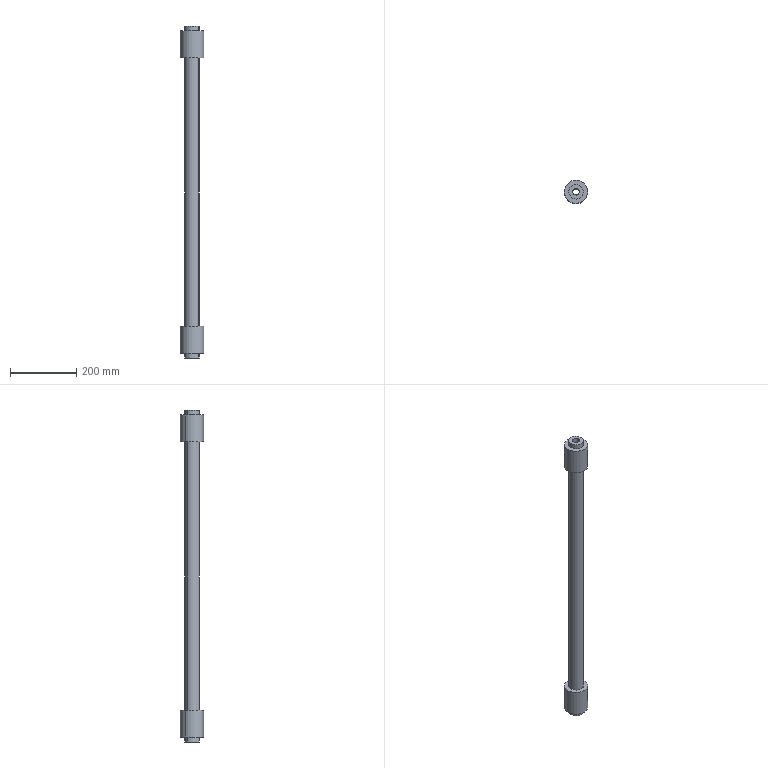Component | SolidWorks | Mandrel-1 | 1 solid | 18 faces | box 70 x 70 x 1000 mm | volume 1589826 mm3 | cylinder 12 | plane 6 | commonest cylinder face diameters 44.189 x6 70 x4 20 x2 | material 45
build123d program:
from build123d import *

# Parameters (mm, degrees)
SKETCH1_R           = 22.094
BOSS_EXTRUDE1_DEPTH = 1000
BOSS_EXTRUDE2_START = 15
SKETCH2_R           = 35
BOSS_EXTRUDE2_DEPTH = 80
SKETCH3_R           = 10
CUT_EXTRUDE1_DEPTH  = 1269.396


with BuildPart() as part:
    # Sketch1 → Boss-Extrude1 (new body)
    with BuildSketch(Plane.XY):
        with Locations((421.144, 598.058)):
            Circle(SKETCH1_R)
    extrude(amount=BOSS_EXTRUDE1_DEPTH)

    # Sketch2 → Boss-Extrude2 (add)
    with BuildSketch(Plane.XY.offset(BOSS_EXTRUDE2_START)):
        with Locations((421.144, 598.058)):
            Circle(SKETCH2_R)
    boss_extrude2 = extrude(amount=BOSS_EXTRUDE2_DEPTH)

    # Mirror1: Boss-Extrude2 across plane
    add(boss_extrude2.mirror(Plane.XY.offset(500)))

    # Sketch3 → Cut-Extrude1 (cut, through all)
    with BuildSketch(Plane(origin=(0, 0, 0), x_dir=(-1, 0, 0), z_dir=(0, 0, -1))):
        with Locations((-421.144, 598.058)):
            Circle(SKETCH3_R)
    extrude(amount=-CUT_EXTRUDE1_DEPTH, mode=Mode.SUBTRACT)


solid = part.part

# Placed as in the assembly
solid = solid.moved(Location((100, 0, -5), (0, 0, 0)))
STEP:
#1=COLOUR_RGB('',0.7922,0.8196,0.9333);
#2=FILL_AREA_STYLE_COLOUR('',#1);
#3=FILL_AREA_STYLE('',(#2));
#4=SURFACE_STYLE_FILL_AREA(#3);
#5=SURFACE_SIDE_STYLE('',(#4));
#6=SURFACE_STYLE_USAGE(.BOTH.,#5);
#7=PRESENTATION_STYLE_ASSIGNMENT((#6));
#8=CARTESIAN_POINT('',(20.191,23.766,39.173));
#9=VERTEX_POINT('',#8);
#10=CARTESIAN_POINT('',(20.844,23.325,39.173));
#11=VERTEX_POINT('',#10);
#12=CARTESIAN_POINT('',(20.517,23.546,39.173));
#13=DIRECTION('',(-0.,0.,-1.));
#14=DIRECTION('',(0.8284,-0.5601,0.));
#15=AXIS2_PLACEMENT_3D('',#12,#13,#14);
#16=CIRCLE('',#15,0.3937);
#17=EDGE_CURVE('',#9,#11,#16,.T.);
#18=ORIENTED_EDGE('',*,*,#17,.F.);
#19=CARTESIAN_POINT('',(20.191,23.766,-0.1969));
#20=VERTEX_POINT('',#19);
#21=CARTESIAN_POINT('',(20.191,23.766,39.173));
#22=DIRECTION('',(-0.,0.,-1.));
#23=VECTOR('',#22,39.37);
#24=LINE('',#21,#23);
#25=EDGE_CURVE('',#9,#20,#24,.T.);
#26=ORIENTED_EDGE('',*,*,#25,.T.);
#27=CARTESIAN_POINT('',(20.844,23.325,-0.1969));
#28=VERTEX_POINT('',#27);
#29=CARTESIAN_POINT('',(20.517,23.546,-0.1969));
#30=DIRECTION('',(-0.,0.,-1.));
#31=DIRECTION('',(0.8284,-0.5601,0.));
#32=AXIS2_PLACEMENT_3D('',#29,#30,#31);
#33=CIRCLE('',#32,0.3937);
#34=EDGE_CURVE('',#20,#28,#33,.T.);
#35=ORIENTED_EDGE('',*,*,#34,.T.);
#36=CARTESIAN_POINT('',(20.844,23.325,39.173));
#37=DIRECTION('',(-0.,0.,-1.));
#38=VECTOR('',#37,39.37);
#39=LINE('',#36,#38);
#40=EDGE_CURVE('',#11,#28,#39,.T.);
#41=ORIENTED_EDGE('',*,*,#40,.F.);
#42=EDGE_LOOP('',(#18,#26,#35,#41));
#43=FACE_OUTER_BOUND('',#42,.T.);
#44=CARTESIAN_POINT('',(20.517,23.546,39.173));
#45=DIRECTION('',(-0.,0.,-1.));
#46=DIRECTION('',(0.8284,-0.5601,0.));
#47=AXIS2_PLACEMENT_3D('',#44,#45,#46);
#48=CYLINDRICAL_SURFACE('',#47,0.3937);
#49=ADVANCED_FACE('',(#43),#48,.F.);
#50=CARTESIAN_POINT('',(19.797,24.033,39.173));
#51=VERTEX_POINT('',#50);
#52=CARTESIAN_POINT('',(21.238,23.058,39.173));
#53=VERTEX_POINT('',#52);
#54=CARTESIAN_POINT('',(20.517,23.546,39.173));
#55=DIRECTION('',(0.,-0.,1.));
#56=DIRECTION('',(-0.8284,0.5601,0.));
#57=AXIS2_PLACEMENT_3D('',#54,#55,#56);
#58=CIRCLE('',#57,0.8699);
#59=EDGE_CURVE('',#51,#53,#58,.T.);
#60=ORIENTED_EDGE('',*,*,#59,.F.);
#61=CARTESIAN_POINT('',(19.797,24.033,38.583));
#62=VERTEX_POINT('',#61);
#63=CARTESIAN_POINT('',(19.797,24.033,39.173));
#64=DIRECTION('',(-0.,0.,-1.));
#65=VECTOR('',#64,39.37);
#66=LINE('',#63,#65);
#67=EDGE_CURVE('',#51,#62,#66,.T.);
#68=ORIENTED_EDGE('',*,*,#67,.T.);
#69=CARTESIAN_POINT('',(21.238,23.058,38.583));
#70=VERTEX_POINT('',#69);
#71=CARTESIAN_POINT('',(20.517,23.546,38.583));
#72=DIRECTION('',(-0.,0.,-1.));
#73=DIRECTION('',(0.8284,-0.5601,0.));
#74=AXIS2_PLACEMENT_3D('',#71,#72,#73);
#75=CIRCLE('',#74,0.8699);
#76=EDGE_CURVE('',#70,#62,#75,.T.);
#77=ORIENTED_EDGE('',*,*,#76,.F.);
#78=CARTESIAN_POINT('',(21.238,23.058,39.173));
#79=DIRECTION('',(-0.,0.,-1.));
#80=VECTOR('',#79,39.37);
#81=LINE('',#78,#80);
#82=EDGE_CURVE('',#53,#70,#81,.T.);
#83=ORIENTED_EDGE('',*,*,#82,.F.);
#84=EDGE_LOOP('',(#60,#68,#77,#83));
#85=FACE_OUTER_BOUND('',#84,.T.);
#86=CARTESIAN_POINT('',(20.517,23.546,39.173));
#87=DIRECTION('',(-0.,0.,-1.));
#88=DIRECTION('',(0.8284,-0.5601,0.));
#89=AXIS2_PLACEMENT_3D('',#86,#87,#88);
#90=CYLINDRICAL_SURFACE('',#89,0.8699);
#91=ADVANCED_FACE('',(#85),#90,.T.);
#92=CARTESIAN_POINT('',(19.376,24.317,35.433));
#93=VERTEX_POINT('',#92);
#94=CARTESIAN_POINT('',(21.659,22.774,35.433));
#95=VERTEX_POINT('',#94);
#96=CARTESIAN_POINT('',(20.517,23.546,35.433));
#97=DIRECTION('',(0.,-0.,1.));
#98=DIRECTION('',(-0.8284,0.5601,0.));
#99=AXIS2_PLACEMENT_3D('',#96,#97,#98);
#100=CIRCLE('',#99,1.378);
#101=EDGE_CURVE('',#93,#95,#100,.T.);
#102=ORIENTED_EDGE('',*,*,#101,.T.);
#103=CARTESIAN_POINT('',(21.659,22.774,38.583));
#104=VERTEX_POINT('',#103);
#105=CARTESIAN_POINT('',(21.659,22.774,35.433));
#106=DIRECTION('',(0.,-0.,1.));
#107=VECTOR('',#106,39.37);
#108=LINE('',#105,#107);
#109=EDGE_CURVE('',#95,#104,#108,.T.);
#110=ORIENTED_EDGE('',*,*,#109,.T.);
#111=CARTESIAN_POINT('',(19.376,24.317,38.583));
#112=VERTEX_POINT('',#111);
#113=CARTESIAN_POINT('',(20.517,23.546,38.583));
#114=DIRECTION('',(0.,-0.,1.));
#115=DIRECTION('',(-0.8284,0.5601,0.));
#116=AXIS2_PLACEMENT_3D('',#113,#114,#115);
#117=CIRCLE('',#116,1.378);
#118=EDGE_CURVE('',#112,#104,#117,.T.);
#119=ORIENTED_EDGE('',*,*,#118,.F.);
#120=CARTESIAN_POINT('',(19.376,24.317,35.433));
#121=DIRECTION('',(0.,-0.,1.));
#122=VECTOR('',#121,39.37);
#123=LINE('',#120,#122);
#124=EDGE_CURVE('',#93,#112,#123,.T.);
#125=ORIENTED_EDGE('',*,*,#124,.F.);
#126=EDGE_LOOP('',(#102,#110,#119,#125));
#127=FACE_OUTER_BOUND('',#126,.T.);
#128=CARTESIAN_POINT('',(20.517,23.546,35.433));
#129=DIRECTION('',(0.,-0.,1.));
#130=DIRECTION('',(-0.8284,0.5601,0.));
#131=AXIS2_PLACEMENT_3D('',#128,#129,#130);
#132=CYLINDRICAL_SURFACE('',#131,1.378);
#133=ADVANCED_FACE('',(#127),#132,.T.);
#134=CARTESIAN_POINT('',(19.797,24.033,0.3937));
#135=VERTEX_POINT('',#134);
#136=CARTESIAN_POINT('',(21.238,23.058,0.3937));
#137=VERTEX_POINT('',#136);
#138=CARTESIAN_POINT('',(20.517,23.546,0.3937));
#139=DIRECTION('',(0.,-0.,1.));
#140=DIRECTION('',(-0.8284,0.5601,0.));
#141=AXIS2_PLACEMENT_3D('',#138,#139,#140);
#142=CIRCLE('',#141,0.8699);
#143=EDGE_CURVE('',#135,#137,#142,.T.);
#144=ORIENTED_EDGE('',*,*,#143,.F.);
#145=CARTESIAN_POINT('',(19.797,24.033,-0.1969));
#146=VERTEX_POINT('',#145);
#147=CARTESIAN_POINT('',(19.797,24.033,39.173));
#148=DIRECTION('',(-0.,0.,-1.));
#149=VECTOR('',#148,39.37);
#150=LINE('',#147,#149);
#151=EDGE_CURVE('',#135,#146,#150,.T.);
#152=ORIENTED_EDGE('',*,*,#151,.T.);
#153=CARTESIAN_POINT('',(21.238,23.058,-0.1969));
#154=VERTEX_POINT('',#153);
#155=CARTESIAN_POINT('',(20.517,23.546,-0.1969));
#156=DIRECTION('',(0.,-0.,1.));
#157=DIRECTION('',(-0.8284,0.5601,0.));
#158=AXIS2_PLACEMENT_3D('',#155,#156,#157);
#159=CIRCLE('',#158,0.8699);
#160=EDGE_CURVE('',#146,#154,#159,.T.);
#161=ORIENTED_EDGE('',*,*,#160,.T.);
#162=CARTESIAN_POINT('',(21.238,23.058,39.173));
#163=DIRECTION('',(-0.,0.,-1.));
#164=VECTOR('',#163,39.37);
#165=LINE('',#162,#164);
#166=EDGE_CURVE('',#137,#154,#165,.T.);
#167=ORIENTED_EDGE('',*,*,#166,.F.);
#168=EDGE_LOOP('',(#144,#152,#161,#167));
#169=FACE_OUTER_BOUND('',#168,.T.);
#170=CARTESIAN_POINT('',(20.517,23.546,39.173));
#171=DIRECTION('',(-0.,0.,-1.));
#172=DIRECTION('',(0.8284,-0.5601,0.));
#173=AXIS2_PLACEMENT_3D('',#170,#171,#172);
#174=CYLINDRICAL_SURFACE('',#173,0.8699);
#175=ADVANCED_FACE('',(#169),#174,.T.);
#176=CARTESIAN_POINT('',(19.376,24.317,3.543));
#177=VERTEX_POINT('',#176);
#178=CARTESIAN_POINT('',(21.659,22.774,3.543));
#179=VERTEX_POINT('',#178);
#180=CARTESIAN_POINT('',(20.517,23.546,3.543));
#181=DIRECTION('',(0.,-0.,1.));
#182=DIRECTION('',(-0.8284,0.5601,0.));
#183=AXIS2_PLACEMENT_3D('',#180,#181,#182);
#184=CIRCLE('',#183,1.378);
#185=EDGE_CURVE('',#177,#179,#184,.T.);
#186=ORIENTED_EDGE('',*,*,#185,.F.);
#187=CARTESIAN_POINT('',(19.376,24.317,0.3937));
#188=VERTEX_POINT('',#187);
#189=CARTESIAN_POINT('',(19.376,24.317,3.543));
#190=DIRECTION('',(-0.,0.,-1.));
#191=VECTOR('',#190,39.37);
#192=LINE('',#189,#191);
#193=EDGE_CURVE('',#177,#188,#192,.T.);
#194=ORIENTED_EDGE('',*,*,#193,.T.);
#195=CARTESIAN_POINT('',(21.659,22.774,0.3937));
#196=VERTEX_POINT('',#195);
#197=CARTESIAN_POINT('',(20.517,23.546,0.3937));
#198=DIRECTION('',(0.,-0.,1.));
#199=DIRECTION('',(-0.8284,0.5601,0.));
#200=AXIS2_PLACEMENT_3D('',#197,#198,#199);
#201=CIRCLE('',#200,1.378);
#202=EDGE_CURVE('',#188,#196,#201,.T.);
#203=ORIENTED_EDGE('',*,*,#202,.T.);
#204=CARTESIAN_POINT('',(21.659,22.774,3.543));
#205=DIRECTION('',(-0.,0.,-1.));
#206=VECTOR('',#205,39.37);
#207=LINE('',#204,#206);
#208=EDGE_CURVE('',#179,#196,#207,.T.);
#209=ORIENTED_EDGE('',*,*,#208,.F.);
#210=EDGE_LOOP('',(#186,#194,#203,#209));
#211=FACE_OUTER_BOUND('',#210,.T.);
#212=CARTESIAN_POINT('',(20.517,23.546,3.543));
#213=DIRECTION('',(-0.,0.,-1.));
#214=DIRECTION('',(0.8284,-0.5601,0.));
#215=AXIS2_PLACEMENT_3D('',#212,#213,#214);
#216=CYLINDRICAL_SURFACE('',#215,1.378);
#217=ADVANCED_FACE('',(#211),#216,.T.);
#218=CARTESIAN_POINT('',(21.238,23.058,35.433));
#219=VERTEX_POINT('',#218);
#220=CARTESIAN_POINT('',(19.797,24.033,35.433));
#221=VERTEX_POINT('',#220);
#222=CARTESIAN_POINT('',(20.517,23.546,35.433));
#223=DIRECTION('',(-0.,0.,-1.));
#224=DIRECTION('',(0.8284,-0.5601,0.));
#225=AXIS2_PLACEMENT_3D('',#222,#223,#224);
#226=CIRCLE('',#225,0.8699);
#227=EDGE_CURVE('',#219,#221,#226,.T.);
#228=ORIENTED_EDGE('',*,*,#227,.T.);
#229=CARTESIAN_POINT('',(19.797,24.033,3.543));
#230=VERTEX_POINT('',#229);
#231=CARTESIAN_POINT('',(19.797,24.033,39.173));
#232=DIRECTION('',(-0.,0.,-1.));
#233=VECTOR('',#232,39.37);
#234=LINE('',#231,#233);
#235=EDGE_CURVE('',#221,#230,#234,.T.);
#236=ORIENTED_EDGE('',*,*,#235,.T.);
#237=CARTESIAN_POINT('',(21.238,23.058,3.543));
#238=VERTEX_POINT('',#237);
#239=CARTESIAN_POINT('',(20.517,23.546,3.543));
#240=DIRECTION('',(0.,-0.,1.));
#241=DIRECTION('',(-0.8284,0.5601,0.));
#242=AXIS2_PLACEMENT_3D('',#239,#240,#241);
#243=CIRCLE('',#242,0.8699);
#244=EDGE_CURVE('',#230,#238,#243,.T.);
#245=ORIENTED_EDGE('',*,*,#244,.T.);
#246=CARTESIAN_POINT('',(21.238,23.058,39.173));
#247=DIRECTION('',(-0.,0.,-1.));
#248=VECTOR('',#247,39.37);
#249=LINE('',#246,#248);
#250=EDGE_CURVE('',#219,#238,#249,.T.);
#251=ORIENTED_EDGE('',*,*,#250,.F.);
#252=EDGE_LOOP('',(#228,#236,#245,#251));
#253=FACE_OUTER_BOUND('',#252,.T.);
#254=CARTESIAN_POINT('',(20.517,23.546,39.173));
#255=DIRECTION('',(-0.,0.,-1.));
#256=DIRECTION('',(0.8284,-0.5601,0.));
#257=AXIS2_PLACEMENT_3D('',#254,#255,#256);
#258=CYLINDRICAL_SURFACE('',#257,0.8699);
#259=ADVANCED_FACE('',(#253),#258,.T.);
#260=ORIENTED_EDGE('',*,*,#235,.F.);
#261=CARTESIAN_POINT('',(20.517,23.546,35.433));
#262=DIRECTION('',(-0.,0.,-1.));
#263=DIRECTION('',(0.8284,-0.5601,0.));
#264=AXIS2_PLACEMENT_3D('',#261,#262,#263);
#265=CIRCLE('',#264,0.8699);
#266=EDGE_CURVE('',#221,#219,#265,.T.);
#267=ORIENTED_EDGE('',*,*,#266,.T.);
#268=ORIENTED_EDGE('',*,*,#250,.T.);
#269=CARTESIAN_POINT('',(20.517,23.546,3.543));
#270=DIRECTION('',(0.,-0.,1.));
#271=DIRECTION('',(-0.8284,0.5601,0.));
#272=AXIS2_PLACEMENT_3D('',#269,#270,#271);
#273=CIRCLE('',#272,0.8699);
#274=EDGE_CURVE('',#238,#230,#273,.T.);
#275=ORIENTED_EDGE('',*,*,#274,.T.);
#276=EDGE_LOOP('',(#260,#267,#268,#275));
#277=FACE_OUTER_BOUND('',#276,.T.);
#278=CARTESIAN_POINT('',(20.517,23.546,39.173));
#279=DIRECTION('',(-0.,0.,-1.));
#280=DIRECTION('',(0.8284,-0.5601,0.));
#281=AXIS2_PLACEMENT_3D('',#278,#279,#280);
#282=CYLINDRICAL_SURFACE('',#281,0.8699);
#283=ADVANCED_FACE('',(#277),#282,.T.);
#284=CARTESIAN_POINT('',(20.517,23.546,3.543));
#285=DIRECTION('',(0.,-0.,1.));
#286=DIRECTION('',(-0.8284,0.5601,0.));
#287=AXIS2_PLACEMENT_3D('',#284,#285,#286);
#288=CIRCLE('',#287,1.378);
#289=EDGE_CURVE('',#179,#177,#288,.T.);
#290=ORIENTED_EDGE('',*,*,#289,.T.);
#291=ORIENTED_EDGE('',*,*,#185,.T.);
#292=EDGE_LOOP('',(#290,#291));
#293=FACE_OUTER_BOUND('',#292,.T.);
#294=ORIENTED_EDGE('',*,*,#274,.F.);
#295=ORIENTED_EDGE('',*,*,#244,.F.);
#296=EDGE_LOOP('',(#294,#295));
#297=FACE_BOUND('',#296,.T.);
#298=CARTESIAN_POINT('',(20.517,23.546,3.543));
#299=DIRECTION('',(0.,-0.,1.));
#300=DIRECTION('',(-0.8284,0.5601,0.));
#301=AXIS2_PLACEMENT_3D('',#298,#299,#300);
#302=PLANE('',#301);
#303=ADVANCED_FACE('',(#293,#297),#302,.T.);
#304=CARTESIAN_POINT('',(20.517,23.546,0.3937));
#305=DIRECTION('',(0.,-0.,1.));
#306=DIRECTION('',(-0.8284,0.5601,0.));
#307=AXIS2_PLACEMENT_3D('',#304,#305,#306);
#308=CIRCLE('',#307,1.378);
#309=EDGE_CURVE('',#196,#188,#308,.T.);
#310=ORIENTED_EDGE('',*,*,#309,.F.);
#311=ORIENTED_EDGE('',*,*,#202,.F.);
#312=EDGE_LOOP('',(#310,#311));
#313=FACE_OUTER_BOUND('',#312,.T.);
#314=CARTESIAN_POINT('',(20.517,23.546,0.3937));
#315=DIRECTION('',(0.,-0.,1.));
#316=DIRECTION('',(-0.8284,0.5601,0.));
#317=AXIS2_PLACEMENT_3D('',#314,#315,#316);
#318=CIRCLE('',#317,0.8699);
#319=EDGE_CURVE('',#137,#135,#318,.T.);
#320=ORIENTED_EDGE('',*,*,#319,.T.);
#321=ORIENTED_EDGE('',*,*,#143,.T.);
#322=EDGE_LOOP('',(#320,#321));
#323=FACE_BOUND('',#322,.T.);
#324=CARTESIAN_POINT('',(20.517,23.546,0.3937));
#325=DIRECTION('',(0.,-0.,1.));
#326=DIRECTION('',(-0.8284,0.5601,0.));
#327=AXIS2_PLACEMENT_3D('',#324,#325,#326);
#328=PLANE('',#327);
#329=ADVANCED_FACE('',(#313,#323),#328,.F.);
#330=ORIENTED_EDGE('',*,*,#193,.F.);
#331=ORIENTED_EDGE('',*,*,#289,.F.);
#332=ORIENTED_EDGE('',*,*,#208,.T.);
#333=ORIENTED_EDGE('',*,*,#309,.T.);
#334=EDGE_LOOP('',(#330,#331,#332,#333));
#335=FACE_OUTER_BOUND('',#334,.T.);
#336=CARTESIAN_POINT('',(20.517,23.546,3.543));
#337=DIRECTION('',(-0.,0.,-1.));
#338=DIRECTION('',(0.8284,-0.5601,0.));
#339=AXIS2_PLACEMENT_3D('',#336,#337,#338);
#340=CYLINDRICAL_SURFACE('',#339,1.378);
#341=ADVANCED_FACE('',(#335),#340,.T.);
#342=CARTESIAN_POINT('',(20.517,23.546,-0.1969));
#343=DIRECTION('',(-0.,0.,-1.));
#344=DIRECTION('',(0.8284,-0.5601,0.));
#345=AXIS2_PLACEMENT_3D('',#342,#343,#344);
#346=CIRCLE('',#345,0.3937);
#347=EDGE_CURVE('',#28,#20,#346,.T.);
#348=ORIENTED_EDGE('',*,*,#347,.F.);
#349=ORIENTED_EDGE('',*,*,#34,.F.);
#350=EDGE_LOOP('',(#348,#349));
#351=FACE_BOUND('',#350,.T.);
#352=CARTESIAN_POINT('',(20.517,23.546,-0.1969));
#353=DIRECTION('',(0.,-0.,1.));
#354=DIRECTION('',(-0.8284,0.5601,0.));
#355=AXIS2_PLACEMENT_3D('',#352,#353,#354);
#356=CIRCLE('',#355,0.8699);
#357=EDGE_CURVE('',#154,#146,#356,.T.);
#358=ORIENTED_EDGE('',*,*,#357,.F.);
#359=ORIENTED_EDGE('',*,*,#160,.F.);
#360=EDGE_LOOP('',(#358,#359));
#361=FACE_OUTER_BOUND('',#360,.T.);
#362=CARTESIAN_POINT('',(20.517,23.546,-0.1969));
#363=DIRECTION('',(0.,-0.,1.));
#364=DIRECTION('',(-0.8284,0.5601,0.));
#365=AXIS2_PLACEMENT_3D('',#362,#363,#364);
#366=PLANE('',#365);
#367=ADVANCED_FACE('',(#351,#361),#366,.F.);
#368=ORIENTED_EDGE('',*,*,#151,.F.);
#369=ORIENTED_EDGE('',*,*,#319,.F.);
#370=ORIENTED_EDGE('',*,*,#166,.T.);
#371=ORIENTED_EDGE('',*,*,#357,.T.);
#372=EDGE_LOOP('',(#368,#369,#370,#371));
#373=FACE_OUTER_BOUND('',#372,.T.);
#374=CARTESIAN_POINT('',(20.517,23.546,39.173));
#375=DIRECTION('',(-0.,0.,-1.));
#376=DIRECTION('',(0.8284,-0.5601,0.));
#377=AXIS2_PLACEMENT_3D('',#374,#375,#376);
#378=CYLINDRICAL_SURFACE('',#377,0.8699);
#379=ADVANCED_FACE('',(#373),#378,.T.);
#380=ORIENTED_EDGE('',*,*,#101,.F.);
#381=CARTESIAN_POINT('',(20.517,23.546,35.433));
#382=DIRECTION('',(0.,-0.,1.));
#383=DIRECTION('',(-0.8284,0.5601,0.));
#384=AXIS2_PLACEMENT_3D('',#381,#382,#383);
#385=CIRCLE('',#384,1.378);
#386=EDGE_CURVE('',#95,#93,#385,.T.);
#387=ORIENTED_EDGE('',*,*,#386,.F.);
#388=EDGE_LOOP('',(#380,#387));
#389=FACE_OUTER_BOUND('',#388,.T.);
#390=ORIENTED_EDGE('',*,*,#227,.F.);
#391=ORIENTED_EDGE('',*,*,#266,.F.);
#392=EDGE_LOOP('',(#390,#391));
#393=FACE_BOUND('',#392,.T.);
#394=CARTESIAN_POINT('',(20.517,23.546,35.433));
#395=DIRECTION('',(-0.,0.,-1.));
#396=DIRECTION('',(-0.8284,0.5601,0.));
#397=AXIS2_PLACEMENT_3D('',#394,#395,#396);
#398=PLANE('',#397);
#399=ADVANCED_FACE('',(#389,#393),#398,.T.);
#400=ORIENTED_EDGE('',*,*,#118,.T.);
#401=CARTESIAN_POINT('',(20.517,23.546,38.583));
#402=DIRECTION('',(0.,-0.,1.));
#403=DIRECTION('',(-0.8284,0.5601,0.));
#404=AXIS2_PLACEMENT_3D('',#401,#402,#403);
#405=CIRCLE('',#404,1.378);
#406=EDGE_CURVE('',#104,#112,#405,.T.);
#407=ORIENTED_EDGE('',*,*,#406,.T.);
#408=EDGE_LOOP('',(#400,#407));
#409=FACE_OUTER_BOUND('',#408,.T.);
#410=ORIENTED_EDGE('',*,*,#76,.T.);
#411=CARTESIAN_POINT('',(20.517,23.546,38.583));
#412=DIRECTION('',(-0.,0.,-1.));
#413=DIRECTION('',(0.8284,-0.5601,0.));
#414=AXIS2_PLACEMENT_3D('',#411,#412,#413);
#415=CIRCLE('',#414,0.8699);
#416=EDGE_CURVE('',#62,#70,#415,.T.);
#417=ORIENTED_EDGE('',*,*,#416,.T.);
#418=EDGE_LOOP('',(#410,#417));
#419=FACE_BOUND('',#418,.T.);
#420=CARTESIAN_POINT('',(20.517,23.546,38.583));
#421=DIRECTION('',(-0.,0.,-1.));
#422=DIRECTION('',(-0.8284,0.5601,0.));
#423=AXIS2_PLACEMENT_3D('',#420,#421,#422);
#424=PLANE('',#423);
#425=ADVANCED_FACE('',(#409,#419),#424,.F.);
#426=ORIENTED_EDGE('',*,*,#109,.F.);
#427=ORIENTED_EDGE('',*,*,#386,.T.);
#428=ORIENTED_EDGE('',*,*,#124,.T.);
#429=ORIENTED_EDGE('',*,*,#406,.F.);
#430=EDGE_LOOP('',(#426,#427,#428,#429));
#431=FACE_OUTER_BOUND('',#430,.T.);
#432=CARTESIAN_POINT('',(20.517,23.546,35.433));
#433=DIRECTION('',(0.,-0.,1.));
#434=DIRECTION('',(-0.8284,0.5601,0.));
#435=AXIS2_PLACEMENT_3D('',#432,#433,#434);
#436=CYLINDRICAL_SURFACE('',#435,1.378);
#437=ADVANCED_FACE('',(#431),#436,.T.);
#438=CARTESIAN_POINT('',(20.517,23.546,39.173));
#439=DIRECTION('',(-0.,0.,-1.));
#440=DIRECTION('',(0.8284,-0.5601,0.));
#441=AXIS2_PLACEMENT_3D('',#438,#439,#440);
#442=CIRCLE('',#441,0.3937);
#443=EDGE_CURVE('',#11,#9,#442,.T.);
#444=ORIENTED_EDGE('',*,*,#443,.T.);
#445=ORIENTED_EDGE('',*,*,#17,.T.);
#446=EDGE_LOOP('',(#444,#445));
#447=FACE_BOUND('',#446,.T.);
#448=CARTESIAN_POINT('',(20.517,23.546,39.173));
#449=DIRECTION('',(0.,-0.,1.));
#450=DIRECTION('',(-0.8284,0.5601,0.));
#451=AXIS2_PLACEMENT_3D('',#448,#449,#450);
#452=CIRCLE('',#451,0.8699);
#453=EDGE_CURVE('',#53,#51,#452,.T.);
#454=ORIENTED_EDGE('',*,*,#453,.T.);
#455=ORIENTED_EDGE('',*,*,#59,.T.);
#456=EDGE_LOOP('',(#454,#455));
#457=FACE_OUTER_BOUND('',#456,.T.);
#458=CARTESIAN_POINT('',(20.517,23.546,39.173));
#459=DIRECTION('',(0.,-0.,1.));
#460=DIRECTION('',(-0.8284,0.5601,0.));
#461=AXIS2_PLACEMENT_3D('',#458,#459,#460);
#462=PLANE('',#461);
#463=ADVANCED_FACE('',(#447,#457),#462,.T.);
#464=ORIENTED_EDGE('',*,*,#67,.F.);
#465=ORIENTED_EDGE('',*,*,#453,.F.);
#466=ORIENTED_EDGE('',*,*,#82,.T.);
#467=ORIENTED_EDGE('',*,*,#416,.F.);
#468=EDGE_LOOP('',(#464,#465,#466,#467));
#469=FACE_OUTER_BOUND('',#468,.T.);
#470=CARTESIAN_POINT('',(20.517,23.546,39.173));
#471=DIRECTION('',(-0.,0.,-1.));
#472=DIRECTION('',(0.8284,-0.5601,0.));
#473=AXIS2_PLACEMENT_3D('',#470,#471,#472);
#474=CYLINDRICAL_SURFACE('',#473,0.8699);
#475=ADVANCED_FACE('',(#469),#474,.T.);
#476=ORIENTED_EDGE('',*,*,#25,.F.);
#477=ORIENTED_EDGE('',*,*,#443,.F.);
#478=ORIENTED_EDGE('',*,*,#40,.T.);
#479=ORIENTED_EDGE('',*,*,#347,.T.);
#480=EDGE_LOOP('',(#476,#477,#478,#479));
#481=FACE_OUTER_BOUND('',#480,.T.);
#482=CARTESIAN_POINT('',(20.517,23.546,39.173));
#483=DIRECTION('',(-0.,0.,-1.));
#484=DIRECTION('',(0.8284,-0.5601,0.));
#485=AXIS2_PLACEMENT_3D('',#482,#483,#484);
#486=CYLINDRICAL_SURFACE('',#485,0.3937);
#487=ADVANCED_FACE('',(#481),#486,.F.);
#488=CLOSED_SHELL('',(#49,#91,#133,#175,#217,#259,#283,#303,#329,#341,#367,#379,#399,#425,#437,#463,#475,#487));
#489=MANIFOLD_SOLID_BREP('',#488);
#490=STYLED_ITEM('',(#7),#489);
#491=(LENGTH_UNIT()NAMED_UNIT(*)SI_UNIT($,.METRE.));
#492=LENGTH_MEASURE_WITH_UNIT(LENGTH_MEASURE(0.0254),#491);
#493=DIMENSIONAL_EXPONENTS(1.,0.,0.,0.,0.,0.,0.);
#494=(CONVERSION_BASED_UNIT('',#492)LENGTH_UNIT()NAMED_UNIT(#493));
#495=UNCERTAINTY_MEASURE_WITH_UNIT(LENGTH_MEASURE(0.00001),#494,'','');
#496=(NAMED_UNIT(*)PLANE_ANGLE_UNIT()SI_UNIT($,.RADIAN.));
#497=(NAMED_UNIT(*)SI_UNIT($,.STERADIAN.)SOLID_ANGLE_UNIT());
#498=(GEOMETRIC_REPRESENTATION_CONTEXT(3)GLOBAL_UNCERTAINTY_ASSIGNED_CONTEXT((#495))GLOBAL_UNIT_ASSIGNED_CONTEXT((#494,#496,#497))REPRESENTATION_CONTEXT('',''));
#499=MECHANICAL_DESIGN_GEOMETRIC_PRESENTATION_REPRESENTATION('',(#490),#498);
#500=CARTESIAN_POINT('',(0.,0.,0.));
#501=DIRECTION('',(0.,0.,1.));
#502=DIRECTION('',(1.,0.,0.));
#503=AXIS2_PLACEMENT_3D('',#500,#501,#502);
#504=(LENGTH_UNIT()NAMED_UNIT(*)SI_UNIT($,.METRE.));
#505=LENGTH_MEASURE_WITH_UNIT(LENGTH_MEASURE(0.0254),#504);
#506=DIMENSIONAL_EXPONENTS(1.,0.,0.,0.,0.,0.,0.);
#507=(CONVERSION_BASED_UNIT('',#505)LENGTH_UNIT()NAMED_UNIT(#506));
#508=UNCERTAINTY_MEASURE_WITH_UNIT(LENGTH_MEASURE(0.00001),#507,'','');
#509=(NAMED_UNIT(*)PLANE_ANGLE_UNIT()SI_UNIT($,.RADIAN.));
#510=(NAMED_UNIT(*)SI_UNIT($,.STERADIAN.)SOLID_ANGLE_UNIT());
#511=(GEOMETRIC_REPRESENTATION_CONTEXT(3)GLOBAL_UNCERTAINTY_ASSIGNED_CONTEXT((#508))GLOBAL_UNIT_ASSIGNED_CONTEXT((#507,#509,#510))REPRESENTATION_CONTEXT('',''));
#512=ADVANCED_BREP_SHAPE_REPRESENTATION('',(#489,#503),#511);
#513=PRESENTATION_LAYER_ASSIGNMENT('','',(#490));